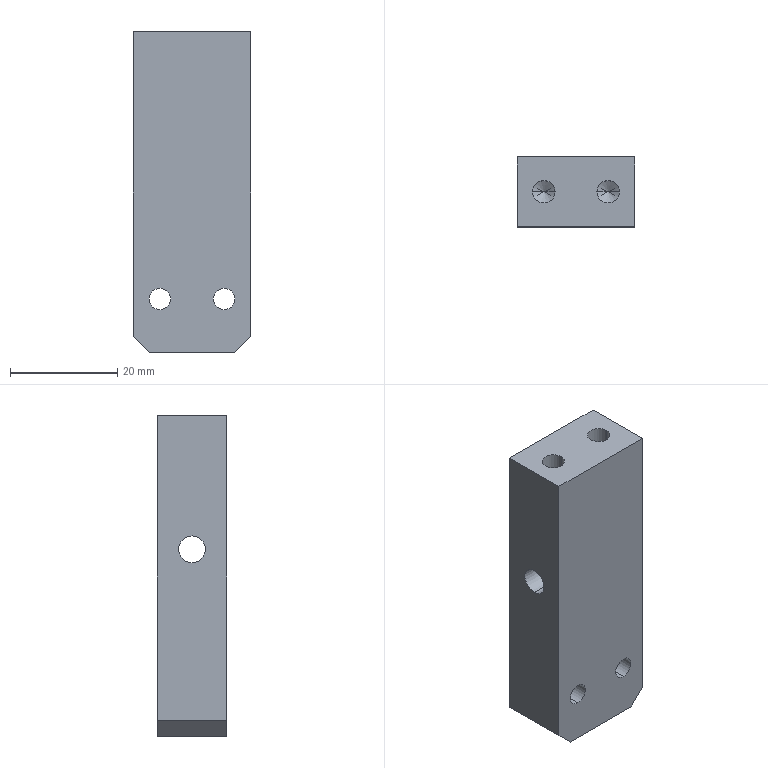Component | SolidWorks | A47-1 | 1 solid | 22 faces | box 22 x 13 x 60 mm | volume 15929 mm3 | cylinder 10 | plane 8 | cone 4 | commonest cylinder face diameters 4.2 x4 4 x4 5 x2 | material S136
build123d program:
from build123d import *

# Parameters (mm, degrees)
SKETCH1_W             = 60
SKETCH1_H             = 13
BOSS_EXTRUDE1_DEPTH   = 11
M5_TAPPED_HOLE3_D     = 5
M4_TAPPED_HOLE1_D     = 4
CHAMFER2_SIZE         = 3
M5_TAPPED_HOLE2_D     = 4.2
M5_TAPPED_HOLE2_DEPTH = 12.4
M5_TAPPED_HOLE2_TIP   = 1.262


with BuildPart() as part:
    # Sketch1 → Boss-Extrude1 (new, symmetric)
    with BuildSketch(Plane(origin=(0, 0, 0), x_dir=(0, 0, -1), z_dir=(1, 0, 0))):
        Rectangle(SKETCH1_W, SKETCH1_H)
    extrude(amount=BOSS_EXTRUDE1_DEPTH, both=True)

    # M5 Tapped Hole3 (through all)
    with Locations(Plane(origin=(11, 0, 0), x_dir=(0, 0, -1), z_dir=(1, 0, 0))):
        with Locations((-5, 0)):
            Hole(M5_TAPPED_HOLE3_D / 2)

    # M4 Tapped Hole1 (through all)
    with Locations(Plane(origin=(0, 6.5, 0), x_dir=(1, 0, 0), z_dir=(0, 1, 0))):
        with Locations((-6, 20), (6, 20)):
            Hole(M4_TAPPED_HOLE1_D / 2)

    # Chamfer2
    chamfer2_edges = [part.edges().sort_by_distance(p)[0] for p in [
        (11, 0, -30),
        (-11, 0, -30),
    ]]
    chamfer(chamfer2_edges, length=CHAMFER2_SIZE)

    # M5 Tapped Hole2
    with Locations(Plane.XY.offset(30)):
        with Locations((-6, 0), (6, 0)):
            Hole(M5_TAPPED_HOLE2_D / 2, depth=M5_TAPPED_HOLE2_DEPTH)
            with Locations((0, 0, -(M5_TAPPED_HOLE2_DEPTH + M5_TAPPED_HOLE2_TIP / 2))):  # 118° drill point
                Cone(0, M5_TAPPED_HOLE2_D / 2, M5_TAPPED_HOLE2_TIP, mode=Mode.SUBTRACT)


solid = part.part

# Placed as in the assembly
solid = solid.moved(Location((-6.351, 25.864, 0), (0, 0, 0)))
STEP:
#1=COLOUR_RGB('',0.7922,0.8196,0.9333);
#2=FILL_AREA_STYLE_COLOUR('',#1);
#3=FILL_AREA_STYLE('',(#2));
#4=SURFACE_STYLE_FILL_AREA(#3);
#5=SURFACE_SIDE_STYLE('',(#4));
#6=SURFACE_STYLE_USAGE(.BOTH.,#5);
#7=PRESENTATION_STYLE_ASSIGNMENT((#6));
#8=CARTESIAN_POINT('',(-0.5689,1.018,0.6929));
#9=VERTEX_POINT('',#8);
#10=CARTESIAN_POINT('',(-0.4036,1.018,0.6929));
#11=VERTEX_POINT('',#10);
#12=CARTESIAN_POINT('',(-0.4863,1.018,0.6929));
#13=DIRECTION('',(0.,0.,1.));
#14=DIRECTION('',(1.,0.,0.));
#15=AXIS2_PLACEMENT_3D('',#12,#13,#14);
#16=CIRCLE('',#15,0.08268);
#17=EDGE_CURVE('',#9,#11,#16,.T.);
#18=ORIENTED_EDGE('',*,*,#17,.F.);
#19=CARTESIAN_POINT('',(-0.5689,1.018,1.181));
#20=VERTEX_POINT('',#19);
#21=CARTESIAN_POINT('',(-0.5689,1.018,1.181));
#22=DIRECTION('',(0.,0.,1.));
#23=VECTOR('',#22,39.37);
#24=LINE('',#21,#23);
#25=EDGE_CURVE('',#9,#20,#24,.T.);
#26=ORIENTED_EDGE('',*,*,#25,.T.);
#27=CARTESIAN_POINT('',(-0.4036,1.018,1.181));
#28=VERTEX_POINT('',#27);
#29=CARTESIAN_POINT('',(-0.4863,1.018,1.181));
#30=DIRECTION('',(0.,0.,1.));
#31=DIRECTION('',(1.,0.,0.));
#32=AXIS2_PLACEMENT_3D('',#29,#30,#31);
#33=CIRCLE('',#32,0.08268);
#34=EDGE_CURVE('',#20,#28,#33,.T.);
#35=ORIENTED_EDGE('',*,*,#34,.T.);
#36=CARTESIAN_POINT('',(-0.4036,1.018,1.181));
#37=DIRECTION('',(0.,0.,1.));
#38=VECTOR('',#37,39.37);
#39=LINE('',#36,#38);
#40=EDGE_CURVE('',#11,#28,#39,.T.);
#41=ORIENTED_EDGE('',*,*,#40,.F.);
#42=EDGE_LOOP('',(#18,#26,#35,#41));
#43=FACE_OUTER_BOUND('',#42,.T.);
#44=CARTESIAN_POINT('',(-0.4863,1.018,1.181));
#45=DIRECTION('',(0.,0.,1.));
#46=DIRECTION('',(1.,0.,0.));
#47=AXIS2_PLACEMENT_3D('',#44,#45,#46);
#48=CYLINDRICAL_SURFACE('',#47,0.08268);
#49=ADVANCED_FACE('',(#43),#48,.F.);
#50=CARTESIAN_POINT('',(-0.4863,1.018,0.6432));
#51=VERTEX_POINT('',#50);
#52=CARTESIAN_POINT('',(-0.4036,1.018,0.6929));
#53=DIRECTION('',(0.8572,0.,0.515));
#54=VECTOR('',#53,39.37);
#55=LINE('',#52,#54);
#56=EDGE_CURVE('',#51,#11,#55,.T.);
#57=ORIENTED_EDGE('',*,*,#56,.F.);
#58=CARTESIAN_POINT('',(-0.5689,1.018,0.6929));
#59=DIRECTION('',(-0.8572,0.,0.515));
#60=VECTOR('',#59,39.37);
#61=LINE('',#58,#60);
#62=EDGE_CURVE('',#51,#9,#61,.T.);
#63=ORIENTED_EDGE('',*,*,#62,.T.);
#64=ORIENTED_EDGE('',*,*,#17,.T.);
#65=EDGE_LOOP('',(#57,#63,#64));
#66=FACE_OUTER_BOUND('',#65,.T.);
#67=CARTESIAN_POINT('',(-0.4863,1.018,0.6929));
#68=DIRECTION('',(0.,0.,1.));
#69=DIRECTION('',(1.,0.,0.));
#70=AXIS2_PLACEMENT_3D('',#67,#68,#69);
#71=CONICAL_SURFACE('',#70,0.08268,1.03);
#72=ADVANCED_FACE('',(#66),#71,.F.);
#73=CARTESIAN_POINT('',(-0.09649,1.018,0.6929));
#74=VERTEX_POINT('',#73);
#75=CARTESIAN_POINT('',(0.06887,1.018,0.6929));
#76=VERTEX_POINT('',#75);
#77=CARTESIAN_POINT('',(-0.01381,1.018,0.6929));
#78=DIRECTION('',(0.,0.,1.));
#79=DIRECTION('',(1.,0.,0.));
#80=AXIS2_PLACEMENT_3D('',#77,#78,#79);
#81=CIRCLE('',#80,0.08268);
#82=EDGE_CURVE('',#74,#76,#81,.T.);
#83=ORIENTED_EDGE('',*,*,#82,.F.);
#84=CARTESIAN_POINT('',(-0.09649,1.018,1.181));
#85=VERTEX_POINT('',#84);
#86=CARTESIAN_POINT('',(-0.09649,1.018,1.181));
#87=DIRECTION('',(0.,0.,1.));
#88=VECTOR('',#87,39.37);
#89=LINE('',#86,#88);
#90=EDGE_CURVE('',#74,#85,#89,.T.);
#91=ORIENTED_EDGE('',*,*,#90,.T.);
#92=CARTESIAN_POINT('',(0.06887,1.018,1.181));
#93=VERTEX_POINT('',#92);
#94=CARTESIAN_POINT('',(-0.01381,1.018,1.181));
#95=DIRECTION('',(0.,0.,1.));
#96=DIRECTION('',(1.,0.,0.));
#97=AXIS2_PLACEMENT_3D('',#94,#95,#96);
#98=CIRCLE('',#97,0.08268);
#99=EDGE_CURVE('',#85,#93,#98,.T.);
#100=ORIENTED_EDGE('',*,*,#99,.T.);
#101=CARTESIAN_POINT('',(0.06887,1.018,1.181));
#102=DIRECTION('',(0.,0.,1.));
#103=VECTOR('',#102,39.37);
#104=LINE('',#101,#103);
#105=EDGE_CURVE('',#76,#93,#104,.T.);
#106=ORIENTED_EDGE('',*,*,#105,.F.);
#107=EDGE_LOOP('',(#83,#91,#100,#106));
#108=FACE_OUTER_BOUND('',#107,.T.);
#109=CARTESIAN_POINT('',(-0.01381,1.018,1.181));
#110=DIRECTION('',(0.,0.,1.));
#111=DIRECTION('',(1.,0.,0.));
#112=AXIS2_PLACEMENT_3D('',#109,#110,#111);
#113=CYLINDRICAL_SURFACE('',#112,0.08268);
#114=ADVANCED_FACE('',(#108),#113,.F.);
#115=CARTESIAN_POINT('',(-0.01381,1.018,0.6432));
#116=VERTEX_POINT('',#115);
#117=CARTESIAN_POINT('',(0.06887,1.018,0.6929));
#118=DIRECTION('',(0.8572,0.,0.515));
#119=VECTOR('',#118,39.37);
#120=LINE('',#117,#119);
#121=EDGE_CURVE('',#116,#76,#120,.T.);
#122=ORIENTED_EDGE('',*,*,#121,.F.);
#123=CARTESIAN_POINT('',(-0.09649,1.018,0.6929));
#124=DIRECTION('',(-0.8572,0.,0.515));
#125=VECTOR('',#124,39.37);
#126=LINE('',#123,#125);
#127=EDGE_CURVE('',#116,#74,#126,.T.);
#128=ORIENTED_EDGE('',*,*,#127,.T.);
#129=ORIENTED_EDGE('',*,*,#82,.T.);
#130=EDGE_LOOP('',(#122,#128,#129));
#131=FACE_OUTER_BOUND('',#130,.T.);
#132=CARTESIAN_POINT('',(-0.01381,1.018,0.6929));
#133=DIRECTION('',(0.,0.,1.));
#134=DIRECTION('',(1.,0.,0.));
#135=AXIS2_PLACEMENT_3D('',#132,#133,#134);
#136=CONICAL_SURFACE('',#135,0.08268,1.03);
#137=ADVANCED_FACE('',(#131),#136,.F.);
#138=CARTESIAN_POINT('',(-0.4863,0.7624,-0.8661));
#139=VERTEX_POINT('',#138);
#140=CARTESIAN_POINT('',(-0.4863,0.7624,-0.7087));
#141=VERTEX_POINT('',#140);
#142=CARTESIAN_POINT('',(-0.4863,0.7624,-0.7874));
#143=DIRECTION('',(0.,1.,0.));
#144=DIRECTION('',(0.,0.,1.));
#145=AXIS2_PLACEMENT_3D('',#142,#143,#144);
#146=CIRCLE('',#145,0.07874);
#147=EDGE_CURVE('',#139,#141,#146,.T.);
#148=ORIENTED_EDGE('',*,*,#147,.F.);
#149=CARTESIAN_POINT('',(-0.4863,1.274,-0.8661));
#150=VERTEX_POINT('',#149);
#151=CARTESIAN_POINT('',(-0.4863,1.274,-0.8661));
#152=DIRECTION('',(0.,1.,0.));
#153=VECTOR('',#152,39.37);
#154=LINE('',#151,#153);
#155=EDGE_CURVE('',#139,#150,#154,.T.);
#156=ORIENTED_EDGE('',*,*,#155,.T.);
#157=CARTESIAN_POINT('',(-0.4863,1.274,-0.7087));
#158=VERTEX_POINT('',#157);
#159=CARTESIAN_POINT('',(-0.4863,1.274,-0.7874));
#160=DIRECTION('',(0.,1.,0.));
#161=DIRECTION('',(0.,0.,1.));
#162=AXIS2_PLACEMENT_3D('',#159,#160,#161);
#163=CIRCLE('',#162,0.07874);
#164=EDGE_CURVE('',#150,#158,#163,.T.);
#165=ORIENTED_EDGE('',*,*,#164,.T.);
#166=CARTESIAN_POINT('',(-0.4863,1.274,-0.7087));
#167=DIRECTION('',(0.,1.,0.));
#168=VECTOR('',#167,39.37);
#169=LINE('',#166,#168);
#170=EDGE_CURVE('',#141,#158,#169,.T.);
#171=ORIENTED_EDGE('',*,*,#170,.F.);
#172=EDGE_LOOP('',(#148,#156,#165,#171));
#173=FACE_OUTER_BOUND('',#172,.T.);
#174=CARTESIAN_POINT('',(-0.4863,1.274,-0.7874));
#175=DIRECTION('',(0.,1.,0.));
#176=DIRECTION('',(0.,0.,1.));
#177=AXIS2_PLACEMENT_3D('',#174,#175,#176);
#178=CYLINDRICAL_SURFACE('',#177,0.07874);
#179=ADVANCED_FACE('',(#173),#178,.F.);
#180=CARTESIAN_POINT('',(-0.01381,0.7624,-0.8661));
#181=VERTEX_POINT('',#180);
#182=CARTESIAN_POINT('',(-0.01381,0.7624,-0.7087));
#183=VERTEX_POINT('',#182);
#184=CARTESIAN_POINT('',(-0.01381,0.7624,-0.7874));
#185=DIRECTION('',(0.,1.,0.));
#186=DIRECTION('',(0.,0.,1.));
#187=AXIS2_PLACEMENT_3D('',#184,#185,#186);
#188=CIRCLE('',#187,0.07874);
#189=EDGE_CURVE('',#181,#183,#188,.T.);
#190=ORIENTED_EDGE('',*,*,#189,.F.);
#191=CARTESIAN_POINT('',(-0.01381,1.274,-0.8661));
#192=VERTEX_POINT('',#191);
#193=CARTESIAN_POINT('',(-0.01381,1.274,-0.8661));
#194=DIRECTION('',(0.,1.,0.));
#195=VECTOR('',#194,39.37);
#196=LINE('',#193,#195);
#197=EDGE_CURVE('',#181,#192,#196,.T.);
#198=ORIENTED_EDGE('',*,*,#197,.T.);
#199=CARTESIAN_POINT('',(-0.01381,1.274,-0.7087));
#200=VERTEX_POINT('',#199);
#201=CARTESIAN_POINT('',(-0.01381,1.274,-0.7874));
#202=DIRECTION('',(0.,1.,0.));
#203=DIRECTION('',(0.,0.,1.));
#204=AXIS2_PLACEMENT_3D('',#201,#202,#203);
#205=CIRCLE('',#204,0.07874);
#206=EDGE_CURVE('',#192,#200,#205,.T.);
#207=ORIENTED_EDGE('',*,*,#206,.T.);
#208=CARTESIAN_POINT('',(-0.01381,1.274,-0.7087));
#209=DIRECTION('',(0.,1.,0.));
#210=VECTOR('',#209,39.37);
#211=LINE('',#208,#210);
#212=EDGE_CURVE('',#183,#200,#211,.T.);
#213=ORIENTED_EDGE('',*,*,#212,.F.);
#214=EDGE_LOOP('',(#190,#198,#207,#213));
#215=FACE_OUTER_BOUND('',#214,.T.);
#216=CARTESIAN_POINT('',(-0.01381,1.274,-0.7874));
#217=DIRECTION('',(0.,1.,0.));
#218=DIRECTION('',(0.,0.,1.));
#219=AXIS2_PLACEMENT_3D('',#216,#217,#218);
#220=CYLINDRICAL_SURFACE('',#219,0.07874);
#221=ADVANCED_FACE('',(#215),#220,.F.);
#222=CARTESIAN_POINT('',(-0.6831,1.018,0.2953));
#223=VERTEX_POINT('',#222);
#224=CARTESIAN_POINT('',(-0.6831,1.018,0.09843));
#225=VERTEX_POINT('',#224);
#226=CARTESIAN_POINT('',(-0.6831,1.018,0.1969));
#227=DIRECTION('',(1.,0.,0.));
#228=DIRECTION('',(0.,0.,-1.));
#229=AXIS2_PLACEMENT_3D('',#226,#227,#228);
#230=CIRCLE('',#229,0.09843);
#231=EDGE_CURVE('',#223,#225,#230,.T.);
#232=ORIENTED_EDGE('',*,*,#231,.F.);
#233=CARTESIAN_POINT('',(0.183,1.018,0.2953));
#234=VERTEX_POINT('',#233);
#235=CARTESIAN_POINT('',(0.183,1.018,0.2953));
#236=DIRECTION('',(1.,0.,0.));
#237=VECTOR('',#236,39.37);
#238=LINE('',#235,#237);
#239=EDGE_CURVE('',#223,#234,#238,.T.);
#240=ORIENTED_EDGE('',*,*,#239,.T.);
#241=CARTESIAN_POINT('',(0.183,1.018,0.09843));
#242=VERTEX_POINT('',#241);
#243=CARTESIAN_POINT('',(0.183,1.018,0.1969));
#244=DIRECTION('',(1.,0.,0.));
#245=DIRECTION('',(0.,0.,-1.));
#246=AXIS2_PLACEMENT_3D('',#243,#244,#245);
#247=CIRCLE('',#246,0.09843);
#248=EDGE_CURVE('',#234,#242,#247,.T.);
#249=ORIENTED_EDGE('',*,*,#248,.T.);
#250=CARTESIAN_POINT('',(0.183,1.018,0.09843));
#251=DIRECTION('',(1.,0.,0.));
#252=VECTOR('',#251,39.37);
#253=LINE('',#250,#252);
#254=EDGE_CURVE('',#225,#242,#253,.T.);
#255=ORIENTED_EDGE('',*,*,#254,.F.);
#256=EDGE_LOOP('',(#232,#240,#249,#255));
#257=FACE_OUTER_BOUND('',#256,.T.);
#258=CARTESIAN_POINT('',(0.183,1.018,0.1969));
#259=DIRECTION('',(1.,0.,0.));
#260=DIRECTION('',(0.,0.,-1.));
#261=AXIS2_PLACEMENT_3D('',#258,#259,#260);
#262=CYLINDRICAL_SURFACE('',#261,0.09843);
#263=ADVANCED_FACE('',(#257),#262,.F.);
#264=CARTESIAN_POINT('',(0.06493,0.7624,-1.181));
#265=VERTEX_POINT('',#264);
#266=CARTESIAN_POINT('',(-0.565,0.7624,-1.181));
#267=VERTEX_POINT('',#266);
#268=CARTESIAN_POINT('',(0.183,0.7624,-1.181));
#269=DIRECTION('',(-1.,0.,0.));
#270=VECTOR('',#269,39.37);
#271=LINE('',#268,#270);
#272=EDGE_CURVE('',#265,#267,#271,.T.);
#273=ORIENTED_EDGE('',*,*,#272,.T.);
#274=CARTESIAN_POINT('',(-0.565,1.274,-1.181));
#275=VERTEX_POINT('',#274);
#276=CARTESIAN_POINT('',(-0.565,1.274,-1.181));
#277=DIRECTION('',(0.,1.,-0.));
#278=VECTOR('',#277,39.37);
#279=LINE('',#276,#278);
#280=EDGE_CURVE('',#267,#275,#279,.T.);
#281=ORIENTED_EDGE('',*,*,#280,.T.);
#282=CARTESIAN_POINT('',(0.06493,1.274,-1.181));
#283=VERTEX_POINT('',#282);
#284=CARTESIAN_POINT('',(0.183,1.274,-1.181));
#285=DIRECTION('',(-1.,0.,0.));
#286=VECTOR('',#285,39.37);
#287=LINE('',#284,#286);
#288=EDGE_CURVE('',#283,#275,#287,.T.);
#289=ORIENTED_EDGE('',*,*,#288,.F.);
#290=CARTESIAN_POINT('',(0.06493,0.7624,-1.181));
#291=DIRECTION('',(0.,-1.,0.));
#292=VECTOR('',#291,39.37);
#293=LINE('',#290,#292);
#294=EDGE_CURVE('',#283,#265,#293,.T.);
#295=ORIENTED_EDGE('',*,*,#294,.T.);
#296=EDGE_LOOP('',(#273,#281,#289,#295));
#297=FACE_OUTER_BOUND('',#296,.T.);
#298=CARTESIAN_POINT('',(0.183,1.274,-1.181));
#299=DIRECTION('',(0.,0.,1.));
#300=DIRECTION('',(0.,-1.,0.));
#301=AXIS2_PLACEMENT_3D('',#298,#299,#300);
#302=PLANE('',#301);
#303=ADVANCED_FACE('',(#297),#302,.F.);
#304=CARTESIAN_POINT('',(-0.4863,1.274,-0.7874));
#305=DIRECTION('',(0.,1.,0.));
#306=DIRECTION('',(0.,0.,1.));
#307=AXIS2_PLACEMENT_3D('',#304,#305,#306);
#308=CIRCLE('',#307,0.07874);
#309=EDGE_CURVE('',#158,#150,#308,.T.);
#310=ORIENTED_EDGE('',*,*,#309,.F.);
#311=ORIENTED_EDGE('',*,*,#164,.F.);
#312=EDGE_LOOP('',(#310,#311));
#313=FACE_BOUND('',#312,.T.);
#314=CARTESIAN_POINT('',(-0.01381,1.274,-0.7874));
#315=DIRECTION('',(0.,1.,0.));
#316=DIRECTION('',(0.,0.,1.));
#317=AXIS2_PLACEMENT_3D('',#314,#315,#316);
#318=CIRCLE('',#317,0.07874);
#319=EDGE_CURVE('',#200,#192,#318,.T.);
#320=ORIENTED_EDGE('',*,*,#319,.F.);
#321=ORIENTED_EDGE('',*,*,#206,.F.);
#322=EDGE_LOOP('',(#320,#321));
#323=FACE_BOUND('',#322,.T.);
#324=ORIENTED_EDGE('',*,*,#288,.T.);
#325=CARTESIAN_POINT('',(-0.6831,1.274,-1.063));
#326=VERTEX_POINT('',#325);
#327=CARTESIAN_POINT('',(-0.565,1.274,-1.181));
#328=DIRECTION('',(-0.7071,0.,0.7071));
#329=VECTOR('',#328,39.37);
#330=LINE('',#327,#329);
#331=EDGE_CURVE('',#275,#326,#330,.T.);
#332=ORIENTED_EDGE('',*,*,#331,.T.);
#333=CARTESIAN_POINT('',(-0.6831,1.274,1.181));
#334=VERTEX_POINT('',#333);
#335=CARTESIAN_POINT('',(-0.6831,1.274,1.181));
#336=DIRECTION('',(0.,0.,1.));
#337=VECTOR('',#336,39.37);
#338=LINE('',#335,#337);
#339=EDGE_CURVE('',#326,#334,#338,.T.);
#340=ORIENTED_EDGE('',*,*,#339,.T.);
#341=CARTESIAN_POINT('',(0.183,1.274,1.181));
#342=VERTEX_POINT('',#341);
#343=CARTESIAN_POINT('',(0.183,1.274,1.181));
#344=DIRECTION('',(-1.,0.,0.));
#345=VECTOR('',#344,39.37);
#346=LINE('',#343,#345);
#347=EDGE_CURVE('',#342,#334,#346,.T.);
#348=ORIENTED_EDGE('',*,*,#347,.F.);
#349=CARTESIAN_POINT('',(0.183,1.274,-1.063));
#350=VERTEX_POINT('',#349);
#351=CARTESIAN_POINT('',(0.183,1.274,1.181));
#352=DIRECTION('',(0.,0.,1.));
#353=VECTOR('',#352,39.37);
#354=LINE('',#351,#353);
#355=EDGE_CURVE('',#350,#342,#354,.T.);
#356=ORIENTED_EDGE('',*,*,#355,.F.);
#357=CARTESIAN_POINT('',(0.183,1.274,-1.063));
#358=DIRECTION('',(-0.7071,0.,-0.7071));
#359=VECTOR('',#358,39.37);
#360=LINE('',#357,#359);
#361=EDGE_CURVE('',#350,#283,#360,.T.);
#362=ORIENTED_EDGE('',*,*,#361,.T.);
#363=EDGE_LOOP('',(#324,#332,#340,#348,#356,#362));
#364=FACE_OUTER_BOUND('',#363,.T.);
#365=CARTESIAN_POINT('',(0.183,1.274,1.181));
#366=DIRECTION('',(0.,-1.,0.));
#367=DIRECTION('',(0.,0.,-1.));
#368=AXIS2_PLACEMENT_3D('',#365,#366,#367);
#369=PLANE('',#368);
#370=ADVANCED_FACE('',(#313,#323,#364),#369,.F.);
#371=CARTESIAN_POINT('',(-0.4863,1.018,1.181));
#372=DIRECTION('',(0.,0.,1.));
#373=DIRECTION('',(1.,0.,0.));
#374=AXIS2_PLACEMENT_3D('',#371,#372,#373);
#375=CIRCLE('',#374,0.08268);
#376=EDGE_CURVE('',#28,#20,#375,.T.);
#377=ORIENTED_EDGE('',*,*,#376,.F.);
#378=ORIENTED_EDGE('',*,*,#34,.F.);
#379=EDGE_LOOP('',(#377,#378));
#380=FACE_BOUND('',#379,.T.);
#381=CARTESIAN_POINT('',(-0.01381,1.018,1.181));
#382=DIRECTION('',(0.,0.,1.));
#383=DIRECTION('',(1.,0.,0.));
#384=AXIS2_PLACEMENT_3D('',#381,#382,#383);
#385=CIRCLE('',#384,0.08268);
#386=EDGE_CURVE('',#93,#85,#385,.T.);
#387=ORIENTED_EDGE('',*,*,#386,.F.);
#388=ORIENTED_EDGE('',*,*,#99,.F.);
#389=EDGE_LOOP('',(#387,#388));
#390=FACE_BOUND('',#389,.T.);
#391=CARTESIAN_POINT('',(-0.6831,0.7624,1.181));
#392=VERTEX_POINT('',#391);
#393=CARTESIAN_POINT('',(-0.6831,1.274,1.181));
#394=DIRECTION('',(0.,-1.,0.));
#395=VECTOR('',#394,39.37);
#396=LINE('',#393,#395);
#397=EDGE_CURVE('',#334,#392,#396,.T.);
#398=ORIENTED_EDGE('',*,*,#397,.T.);
#399=CARTESIAN_POINT('',(0.183,0.7624,1.181));
#400=VERTEX_POINT('',#399);
#401=CARTESIAN_POINT('',(0.183,0.7624,1.181));
#402=DIRECTION('',(-1.,0.,0.));
#403=VECTOR('',#402,39.37);
#404=LINE('',#401,#403);
#405=EDGE_CURVE('',#400,#392,#404,.T.);
#406=ORIENTED_EDGE('',*,*,#405,.F.);
#407=CARTESIAN_POINT('',(0.183,1.274,1.181));
#408=DIRECTION('',(0.,-1.,0.));
#409=VECTOR('',#408,39.37);
#410=LINE('',#407,#409);
#411=EDGE_CURVE('',#342,#400,#410,.T.);
#412=ORIENTED_EDGE('',*,*,#411,.F.);
#413=ORIENTED_EDGE('',*,*,#347,.T.);
#414=EDGE_LOOP('',(#398,#406,#412,#413));
#415=FACE_OUTER_BOUND('',#414,.T.);
#416=CARTESIAN_POINT('',(0.183,1.274,1.181));
#417=DIRECTION('',(0.,0.,-1.));
#418=DIRECTION('',(-1.,0.,0.));
#419=AXIS2_PLACEMENT_3D('',#416,#417,#418);
#420=PLANE('',#419);
#421=ADVANCED_FACE('',(#380,#390,#415),#420,.F.);
#422=CARTESIAN_POINT('',(-0.4863,0.7624,-0.7874));
#423=DIRECTION('',(0.,1.,0.));
#424=DIRECTION('',(0.,0.,1.));
#425=AXIS2_PLACEMENT_3D('',#422,#423,#424);
#426=CIRCLE('',#425,0.07874);
#427=EDGE_CURVE('',#141,#139,#426,.T.);
#428=ORIENTED_EDGE('',*,*,#427,.T.);
#429=ORIENTED_EDGE('',*,*,#147,.T.);
#430=EDGE_LOOP('',(#428,#429));
#431=FACE_BOUND('',#430,.T.);
#432=CARTESIAN_POINT('',(-0.01381,0.7624,-0.7874));
#433=DIRECTION('',(0.,1.,0.));
#434=DIRECTION('',(0.,0.,1.));
#435=AXIS2_PLACEMENT_3D('',#432,#433,#434);
#436=CIRCLE('',#435,0.07874);
#437=EDGE_CURVE('',#183,#181,#436,.T.);
#438=ORIENTED_EDGE('',*,*,#437,.T.);
#439=ORIENTED_EDGE('',*,*,#189,.T.);
#440=EDGE_LOOP('',(#438,#439));
#441=FACE_BOUND('',#440,.T.);
#442=CARTESIAN_POINT('',(-0.6831,0.7624,-1.063));
#443=VERTEX_POINT('',#442);
#444=CARTESIAN_POINT('',(-0.6831,0.7624,1.181));
#445=DIRECTION('',(0.,0.,-1.));
#446=VECTOR('',#445,39.37);
#447=LINE('',#444,#446);
#448=EDGE_CURVE('',#392,#443,#447,.T.);
#449=ORIENTED_EDGE('',*,*,#448,.T.);
#450=CARTESIAN_POINT('',(-0.565,0.7624,-1.181));
#451=DIRECTION('',(0.7071,0.,-0.7071));
#452=VECTOR('',#451,39.37);
#453=LINE('',#450,#452);
#454=EDGE_CURVE('',#443,#267,#453,.T.);
#455=ORIENTED_EDGE('',*,*,#454,.T.);
#456=ORIENTED_EDGE('',*,*,#272,.F.);
#457=CARTESIAN_POINT('',(0.183,0.7624,-1.063));
#458=VERTEX_POINT('',#457);
#459=CARTESIAN_POINT('',(0.183,0.7624,-1.063));
#460=DIRECTION('',(0.7071,0.,0.7071));
#461=VECTOR('',#460,39.37);
#462=LINE('',#459,#461);
#463=EDGE_CURVE('',#265,#458,#462,.T.);
#464=ORIENTED_EDGE('',*,*,#463,.T.);
#465=CARTESIAN_POINT('',(0.183,0.7624,1.181));
#466=DIRECTION('',(0.,0.,-1.));
#467=VECTOR('',#466,39.37);
#468=LINE('',#465,#467);
#469=EDGE_CURVE('',#400,#458,#468,.T.);
#470=ORIENTED_EDGE('',*,*,#469,.F.);
#471=ORIENTED_EDGE('',*,*,#405,.T.);
#472=EDGE_LOOP('',(#449,#455,#456,#464,#470,#471));
#473=FACE_OUTER_BOUND('',#472,.T.);
#474=CARTESIAN_POINT('',(0.183,0.7624,1.181));
#475=DIRECTION('',(0.,1.,0.));
#476=DIRECTION('',(0.,0.,1.));
#477=AXIS2_PLACEMENT_3D('',#474,#475,#476);
#478=PLANE('',#477);
#479=ADVANCED_FACE('',(#431,#441,#473),#478,.F.);
#480=CARTESIAN_POINT('',(0.183,1.018,0.1969));
#481=DIRECTION('',(1.,0.,0.));
#482=DIRECTION('',(0.,0.,-1.));
#483=AXIS2_PLACEMENT_3D('',#480,#481,#482);
#484=CIRCLE('',#483,0.09843);
#485=EDGE_CURVE('',#242,#234,#484,.T.);
#486=ORIENTED_EDGE('',*,*,#485,.F.);
#487=ORIENTED_EDGE('',*,*,#248,.F.);
#488=EDGE_LOOP('',(#486,#487));
#489=FACE_BOUND('',#488,.T.);
#490=ORIENTED_EDGE('',*,*,#469,.T.);
#491=CARTESIAN_POINT('',(0.183,1.274,-1.063));
#492=DIRECTION('',(0.,1.,-0.));
#493=VECTOR('',#492,39.37);
#494=LINE('',#491,#493);
#495=EDGE_CURVE('',#458,#350,#494,.T.);
#496=ORIENTED_EDGE('',*,*,#495,.T.);
#497=ORIENTED_EDGE('',*,*,#355,.T.);
#498=ORIENTED_EDGE('',*,*,#411,.T.);
#499=EDGE_LOOP('',(#490,#496,#497,#498));
#500=FACE_OUTER_BOUND('',#499,.T.);
#501=CARTESIAN_POINT('',(0.183,1.018,-0.));
#502=DIRECTION('',(1.,0.,0.));
#503=DIRECTION('',(0.,0.,-1.));
#504=AXIS2_PLACEMENT_3D('',#501,#502,#503);
#505=PLANE('',#504);
#506=ADVANCED_FACE('',(#489,#500),#505,.T.);
#507=CARTESIAN_POINT('',(-0.6831,1.018,0.1969));
#508=DIRECTION('',(1.,0.,0.));
#509=DIRECTION('',(0.,0.,-1.));
#510=AXIS2_PLACEMENT_3D('',#507,#508,#509);
#511=CIRCLE('',#510,0.09843);
#512=EDGE_CURVE('',#225,#223,#511,.T.);
#513=ORIENTED_EDGE('',*,*,#512,.T.);
#514=ORIENTED_EDGE('',*,*,#231,.T.);
#515=EDGE_LOOP('',(#513,#514));
#516=FACE_BOUND('',#515,.T.);
#517=ORIENTED_EDGE('',*,*,#339,.F.);
#518=CARTESIAN_POINT('',(-0.6831,1.018,-1.063));
#519=DIRECTION('',(0.,-1.,0.));
#520=VECTOR('',#519,39.37);
#521=LINE('',#518,#520);
#522=EDGE_CURVE('',#326,#443,#521,.T.);
#523=ORIENTED_EDGE('',*,*,#522,.T.);
#524=ORIENTED_EDGE('',*,*,#448,.F.);
#525=ORIENTED_EDGE('',*,*,#397,.F.);
#526=EDGE_LOOP('',(#517,#523,#524,#525));
#527=FACE_OUTER_BOUND('',#526,.T.);
#528=CARTESIAN_POINT('',(-0.6831,1.018,-0.));
#529=DIRECTION('',(1.,0.,0.));
#530=DIRECTION('',(0.,0.,-1.));
#531=AXIS2_PLACEMENT_3D('',#528,#529,#530);
#532=PLANE('',#531);
#533=ADVANCED_FACE('',(#516,#527),#532,.F.);
#534=ORIENTED_EDGE('',*,*,#239,.F.);
#535=ORIENTED_EDGE('',*,*,#512,.F.);
#536=ORIENTED_EDGE('',*,*,#254,.T.);
#537=ORIENTED_EDGE('',*,*,#485,.T.);
#538=EDGE_LOOP('',(#534,#535,#536,#537));
#539=FACE_OUTER_BOUND('',#538,.T.);
#540=CARTESIAN_POINT('',(0.183,1.018,0.1969));
#541=DIRECTION('',(1.,0.,0.));
#542=DIRECTION('',(0.,0.,-1.));
#543=AXIS2_PLACEMENT_3D('',#540,#541,#542);
#544=CYLINDRICAL_SURFACE('',#543,0.09843);
#545=ADVANCED_FACE('',(#539),#544,.F.);
#546=ORIENTED_EDGE('',*,*,#197,.F.);
#547=ORIENTED_EDGE('',*,*,#437,.F.);
#548=ORIENTED_EDGE('',*,*,#212,.T.);
#549=ORIENTED_EDGE('',*,*,#319,.T.);
#550=EDGE_LOOP('',(#546,#547,#548,#549));
#551=FACE_OUTER_BOUND('',#550,.T.);
#552=CARTESIAN_POINT('',(-0.01381,1.274,-0.7874));
#553=DIRECTION('',(0.,1.,0.));
#554=DIRECTION('',(0.,0.,1.));
#555=AXIS2_PLACEMENT_3D('',#552,#553,#554);
#556=CYLINDRICAL_SURFACE('',#555,0.07874);
#557=ADVANCED_FACE('',(#551),#556,.F.);
#558=ORIENTED_EDGE('',*,*,#155,.F.);
#559=ORIENTED_EDGE('',*,*,#427,.F.);
#560=ORIENTED_EDGE('',*,*,#170,.T.);
#561=ORIENTED_EDGE('',*,*,#309,.T.);
#562=EDGE_LOOP('',(#558,#559,#560,#561));
#563=FACE_OUTER_BOUND('',#562,.T.);
#564=CARTESIAN_POINT('',(-0.4863,1.274,-0.7874));
#565=DIRECTION('',(0.,1.,0.));
#566=DIRECTION('',(0.,0.,1.));
#567=AXIS2_PLACEMENT_3D('',#564,#565,#566);
#568=CYLINDRICAL_SURFACE('',#567,0.07874);
#569=ADVANCED_FACE('',(#563),#568,.F.);
#570=ORIENTED_EDGE('',*,*,#454,.F.);
#571=ORIENTED_EDGE('',*,*,#522,.F.);
#572=ORIENTED_EDGE('',*,*,#331,.F.);
#573=ORIENTED_EDGE('',*,*,#280,.F.);
#574=EDGE_LOOP('',(#570,#571,#572,#573));
#575=FACE_OUTER_BOUND('',#574,.T.);
#576=CARTESIAN_POINT('',(-0.565,1.274,-1.181));
#577=DIRECTION('',(0.7071,0.,0.7071));
#578=DIRECTION('',(0.,1.,-0.));
#579=AXIS2_PLACEMENT_3D('',#576,#577,#578);
#580=PLANE('',#579);
#581=ADVANCED_FACE('',(#575),#580,.F.);
#582=ORIENTED_EDGE('',*,*,#463,.F.);
#583=ORIENTED_EDGE('',*,*,#294,.F.);
#584=ORIENTED_EDGE('',*,*,#361,.F.);
#585=ORIENTED_EDGE('',*,*,#495,.F.);
#586=EDGE_LOOP('',(#582,#583,#584,#585));
#587=FACE_OUTER_BOUND('',#586,.T.);
#588=CARTESIAN_POINT('',(0.183,1.018,-1.063));
#589=DIRECTION('',(0.7071,-0.,-0.7071));
#590=DIRECTION('',(0.,-1.,0.));
#591=AXIS2_PLACEMENT_3D('',#588,#589,#590);
#592=PLANE('',#591);
#593=ADVANCED_FACE('',(#587),#592,.T.);
#594=ORIENTED_EDGE('',*,*,#127,.F.);
#595=ORIENTED_EDGE('',*,*,#121,.T.);
#596=CARTESIAN_POINT('',(-0.01381,1.018,0.6929));
#597=DIRECTION('',(0.,0.,1.));
#598=DIRECTION('',(1.,0.,0.));
#599=AXIS2_PLACEMENT_3D('',#596,#597,#598);
#600=CIRCLE('',#599,0.08268);
#601=EDGE_CURVE('',#76,#74,#600,.T.);
#602=ORIENTED_EDGE('',*,*,#601,.T.);
#603=EDGE_LOOP('',(#594,#595,#602));
#604=FACE_OUTER_BOUND('',#603,.T.);
#605=CARTESIAN_POINT('',(-0.01381,1.018,0.6929));
#606=DIRECTION('',(0.,0.,1.));
#607=DIRECTION('',(1.,0.,0.));
#608=AXIS2_PLACEMENT_3D('',#605,#606,#607);
#609=CONICAL_SURFACE('',#608,0.08268,1.03);
#610=ADVANCED_FACE('',(#604),#609,.F.);
#611=ORIENTED_EDGE('',*,*,#90,.F.);
#612=ORIENTED_EDGE('',*,*,#601,.F.);
#613=ORIENTED_EDGE('',*,*,#105,.T.);
#614=ORIENTED_EDGE('',*,*,#386,.T.);
#615=EDGE_LOOP('',(#611,#612,#613,#614));
#616=FACE_OUTER_BOUND('',#615,.T.);
#617=CARTESIAN_POINT('',(-0.01381,1.018,1.181));
#618=DIRECTION('',(0.,0.,1.));
#619=DIRECTION('',(1.,0.,0.));
#620=AXIS2_PLACEMENT_3D('',#617,#618,#619);
#621=CYLINDRICAL_SURFACE('',#620,0.08268);
#622=ADVANCED_FACE('',(#616),#621,.F.);
#623=ORIENTED_EDGE('',*,*,#62,.F.);
#624=ORIENTED_EDGE('',*,*,#56,.T.);
#625=CARTESIAN_POINT('',(-0.4863,1.018,0.6929));
#626=DIRECTION('',(0.,0.,1.));
#627=DIRECTION('',(1.,0.,0.));
#628=AXIS2_PLACEMENT_3D('',#625,#626,#627);
#629=CIRCLE('',#628,0.08268);
#630=EDGE_CURVE('',#11,#9,#629,.T.);
#631=ORIENTED_EDGE('',*,*,#630,.T.);
#632=EDGE_LOOP('',(#623,#624,#631));
#633=FACE_OUTER_BOUND('',#632,.T.);
#634=CARTESIAN_POINT('',(-0.4863,1.018,0.6929));
#635=DIRECTION('',(0.,0.,1.));
#636=DIRECTION('',(1.,0.,0.));
#637=AXIS2_PLACEMENT_3D('',#634,#635,#636);
#638=CONICAL_SURFACE('',#637,0.08268,1.03);
#639=ADVANCED_FACE('',(#633),#638,.F.);
#640=ORIENTED_EDGE('',*,*,#25,.F.);
#641=ORIENTED_EDGE('',*,*,#630,.F.);
#642=ORIENTED_EDGE('',*,*,#40,.T.);
#643=ORIENTED_EDGE('',*,*,#376,.T.);
#644=EDGE_LOOP('',(#640,#641,#642,#643));
#645=FACE_OUTER_BOUND('',#644,.T.);
#646=CARTESIAN_POINT('',(-0.4863,1.018,1.181));
#647=DIRECTION('',(0.,0.,1.));
#648=DIRECTION('',(1.,0.,0.));
#649=AXIS2_PLACEMENT_3D('',#646,#647,#648);
#650=CYLINDRICAL_SURFACE('',#649,0.08268);
#651=ADVANCED_FACE('',(#645),#650,.F.);
#652=CLOSED_SHELL('',(#49,#72,#114,#137,#179,#221,#263,#303,#370,#421,#479,#506,#533,#545,#557,#569,#581,#593,#610,#622,#639,#651));
#653=MANIFOLD_SOLID_BREP('',#652);
#654=STYLED_ITEM('',(#7),#653);
#655=(LENGTH_UNIT()NAMED_UNIT(*)SI_UNIT($,.METRE.));
#656=LENGTH_MEASURE_WITH_UNIT(LENGTH_MEASURE(0.0254),#655);
#657=DIMENSIONAL_EXPONENTS(1.,0.,0.,0.,0.,0.,0.);
#658=(CONVERSION_BASED_UNIT('',#656)LENGTH_UNIT()NAMED_UNIT(#657));
#659=UNCERTAINTY_MEASURE_WITH_UNIT(LENGTH_MEASURE(0.00001),#658,'','');
#660=(NAMED_UNIT(*)PLANE_ANGLE_UNIT()SI_UNIT($,.RADIAN.));
#661=(NAMED_UNIT(*)SI_UNIT($,.STERADIAN.)SOLID_ANGLE_UNIT());
#662=(GEOMETRIC_REPRESENTATION_CONTEXT(3)GLOBAL_UNCERTAINTY_ASSIGNED_CONTEXT((#659))GLOBAL_UNIT_ASSIGNED_CONTEXT((#658,#660,#661))REPRESENTATION_CONTEXT('',''));
#663=MECHANICAL_DESIGN_GEOMETRIC_PRESENTATION_REPRESENTATION('',(#654),#662);
#664=CARTESIAN_POINT('',(0.,0.,0.));
#665=DIRECTION('',(0.,0.,1.));
#666=DIRECTION('',(1.,0.,0.));
#667=AXIS2_PLACEMENT_3D('',#664,#665,#666);
#668=(LENGTH_UNIT()NAMED_UNIT(*)SI_UNIT($,.METRE.));
#669=LENGTH_MEASURE_WITH_UNIT(LENGTH_MEASURE(0.0254),#668);
#670=DIMENSIONAL_EXPONENTS(1.,0.,0.,0.,0.,0.,0.);
#671=(CONVERSION_BASED_UNIT('',#669)LENGTH_UNIT()NAMED_UNIT(#670));
#672=UNCERTAINTY_MEASURE_WITH_UNIT(LENGTH_MEASURE(0.00001),#671,'','');
#673=(NAMED_UNIT(*)PLANE_ANGLE_UNIT()SI_UNIT($,.RADIAN.));
#674=(NAMED_UNIT(*)SI_UNIT($,.STERADIAN.)SOLID_ANGLE_UNIT());
#675=(GEOMETRIC_REPRESENTATION_CONTEXT(3)GLOBAL_UNCERTAINTY_ASSIGNED_CONTEXT((#672))GLOBAL_UNIT_ASSIGNED_CONTEXT((#671,#673,#674))REPRESENTATION_CONTEXT('',''));
#676=ADVANCED_BREP_SHAPE_REPRESENTATION('',(#653,#667),#675);
#677=PRESENTATION_LAYER_ASSIGNMENT('','',(#654));